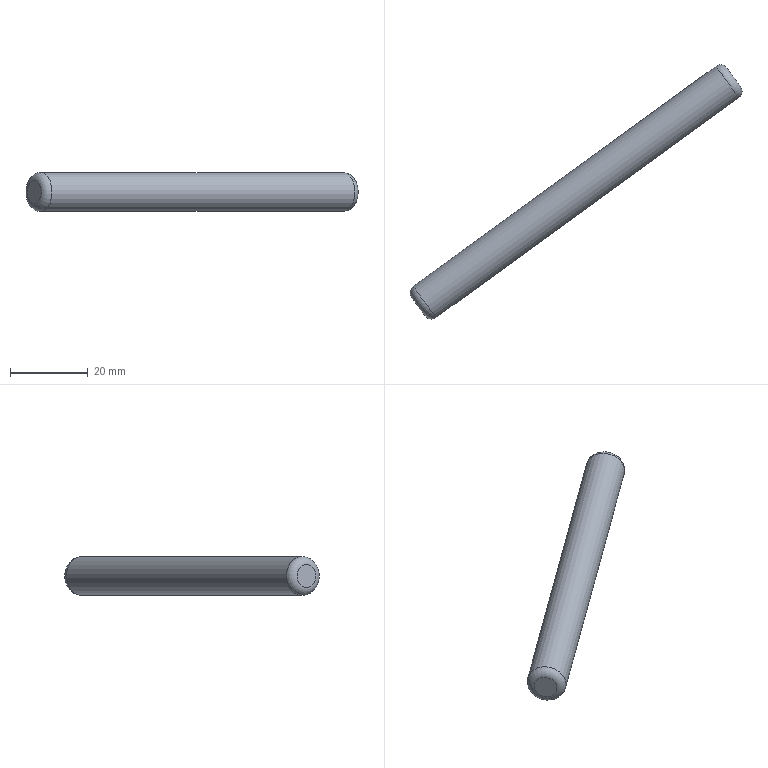Component | NX | CIBIK4 | 1 solid | 5 faces | box 85.19 x 65.28 x 10 mm | volume 7805 mm3 | plane 2 | torus 2 | cylinder 1 | commonest cylinder face diameters 10 x1
STEP:
#1=CARTESIAN_POINT('',(0.,0.,0.));
#2=DIRECTION('',(0.,0.,1.));
#3=DIRECTION('',(1.,0.,0.));
#4=AXIS2_PLACEMENT_3D('',#1,#2,#3);
#5=CARTESIAN_POINT('',(-1267.51,728.811,44.978));
#6=VERTEX_POINT('',#5);
#7=CARTESIAN_POINT('',(-1267.51,728.811,49.978));
#8=DIRECTION('',(0.809,0.5878,0.));
#9=DIRECTION('',(0.,0.,-1.));
#10=AXIS2_PLACEMENT_3D('',#7,#8,#9);
#11=CIRCLE('',#10,5.);
#12=CARTESIAN_POINT('',(-1188.227,786.414,49.978));
#13=DIRECTION('',(-0.809,-0.5878,0.));
#14=DIRECTION('',(0.,0.,1.));
#15=AXIS2_PLACEMENT_3D('',#12,#13,#14);
#16=CYLINDRICAL_SURFACE('',#15,5.);
#17=CARTESIAN_POINT('',(9.425,98.));
#18=DIRECTION('',(-1.,0.));
#19=VECTOR('',#18,1.);
#20=LINE('',#17,#19);
#21=(GEOMETRIC_REPRESENTATION_CONTEXT(2)PARAMETRIC_REPRESENTATION_CONTEXT()REPRESENTATION_CONTEXT('',''));
#22=DEFINITIONAL_REPRESENTATION('',(#20),#21);
#23=PCURVE('',#16,#22);
#24=CARTESIAN_POINT('',(-1267.51,728.811,49.978));
#25=DIRECTION('',(0.809,0.5878,0.));
#26=DIRECTION('',(0.,0.,-1.));
#27=AXIS2_PLACEMENT_3D('',#24,#25,#26);
#28=TOROIDAL_SURFACE('',#27,3.,2.);
#29=CARTESIAN_POINT('',(0.,6.283));
#30=DIRECTION('',(1.,0.));
#31=VECTOR('',#30,1.);
#32=LINE('',#29,#31);
#33=(GEOMETRIC_REPRESENTATION_CONTEXT(2)PARAMETRIC_REPRESENTATION_CONTEXT()REPRESENTATION_CONTEXT('',''));
#34=DEFINITIONAL_REPRESENTATION('',(#32),#33);
#35=PCURVE('',#28,#34);
#36=SURFACE_CURVE('',#11,(#23,#35),.PCURVE_S1.);
#37=EDGE_CURVE('',#6,#6,#36,.T.);
#38=ORIENTED_EDGE('',*,*,#37,.T.);
#39=CARTESIAN_POINT('',(-1189.845,785.238,44.978));
#40=VERTEX_POINT('',#39);
#41=CARTESIAN_POINT('',(-1189.845,785.238,44.978));
#42=CARTESIAN_POINT('',(-1267.51,728.811,44.978));
#43=B_SPLINE_CURVE_WITH_KNOTS('',1,(#41,#42),.UNSPECIFIED.,.F.,.F.,(2,2),(2.,98.),.PIECEWISE_BEZIER_KNOTS.);
#44=CARTESIAN_POINT('',(3.142,0.));
#45=DIRECTION('',(0.,1.));
#46=VECTOR('',#45,1.);
#47=LINE('',#44,#46);
#48=(GEOMETRIC_REPRESENTATION_CONTEXT(2)PARAMETRIC_REPRESENTATION_CONTEXT()REPRESENTATION_CONTEXT('',''));
#49=DEFINITIONAL_REPRESENTATION('',(#47),#48);
#50=PCURVE('',#16,#49);
#51=CARTESIAN_POINT('',(9.425,0.));
#52=DIRECTION('',(0.,1.));
#53=VECTOR('',#52,1.);
#54=LINE('',#51,#53);
#55=(GEOMETRIC_REPRESENTATION_CONTEXT(2)PARAMETRIC_REPRESENTATION_CONTEXT()REPRESENTATION_CONTEXT('',''));
#56=DEFINITIONAL_REPRESENTATION('',(#54),#55);
#57=PCURVE('',#16,#56);
#58=SEAM_CURVE('',#43,(#50,#57),.PCURVE_S1.);
#59=EDGE_CURVE('',#40,#6,#58,.T.);
#60=ORIENTED_EDGE('',*,*,#59,.F.);
#61=CARTESIAN_POINT('',(-1189.845,785.238,49.978));
#62=DIRECTION('',(-0.809,-0.5878,0.));
#63=DIRECTION('',(0.,0.,-1.));
#64=AXIS2_PLACEMENT_3D('',#61,#62,#63);
#65=CIRCLE('',#64,5.);
#66=CARTESIAN_POINT('',(3.142,2.));
#67=DIRECTION('',(1.,0.));
#68=VECTOR('',#67,1.);
#69=LINE('',#66,#68);
#70=(GEOMETRIC_REPRESENTATION_CONTEXT(2)PARAMETRIC_REPRESENTATION_CONTEXT()REPRESENTATION_CONTEXT('',''));
#71=DEFINITIONAL_REPRESENTATION('',(#69),#70);
#72=PCURVE('',#16,#71);
#73=CARTESIAN_POINT('',(-1189.845,785.238,49.978));
#74=DIRECTION('',(0.809,0.5878,0.));
#75=DIRECTION('',(0.,0.,-1.));
#76=AXIS2_PLACEMENT_3D('',#73,#74,#75);
#77=TOROIDAL_SURFACE('',#76,3.,2.);
#78=CARTESIAN_POINT('',(6.283,6.283));
#79=CARTESIAN_POINT('',(6.188,6.283));
#80=CARTESIAN_POINT('',(5.998,6.283));
#81=CARTESIAN_POINT('',(5.712,6.283));
#82=CARTESIAN_POINT('',(5.426,6.283));
#83=CARTESIAN_POINT('',(5.141,6.283));
#84=CARTESIAN_POINT('',(4.855,6.283));
#85=CARTESIAN_POINT('',(4.57,6.283));
#86=CARTESIAN_POINT('',(4.284,6.283));
#87=CARTESIAN_POINT('',(3.998,6.283));
#88=CARTESIAN_POINT('',(3.713,6.283));
#89=CARTESIAN_POINT('',(3.427,6.283));
#90=CARTESIAN_POINT('',(3.142,6.283));
#91=CARTESIAN_POINT('',(2.856,6.283));
#92=CARTESIAN_POINT('',(2.57,6.283));
#93=CARTESIAN_POINT('',(2.285,6.283));
#94=CARTESIAN_POINT('',(1.999,6.283));
#95=CARTESIAN_POINT('',(1.714,6.283));
#96=CARTESIAN_POINT('',(1.428,6.283));
#97=CARTESIAN_POINT('',(1.142,6.283));
#98=CARTESIAN_POINT('',(0.8568,6.283));
#99=CARTESIAN_POINT('',(0.5712,6.283));
#100=CARTESIAN_POINT('',(0.2856,6.283));
#101=CARTESIAN_POINT('',(0.0952,6.283));
#102=CARTESIAN_POINT('',(-0.,6.283));
#103=B_SPLINE_CURVE_WITH_KNOTS('',3,(#78,#79,#80,#81,#82,#83,#84,#85,#86,#87,#88,#89,#90,#91,#92,#93,#94,#95,#96,#97,#98,#99,#100,#101,#102),.UNSPECIFIED.,.F.,.F.,(4,1,1,1,1,1,1,1,1,1,1,1,1,1,1,1,1,1,1,1,1,1,4),(0.,0.2856,0.5712,0.8568,1.142,1.428,1.714,1.999,2.285,2.57,2.856,3.142,3.427,3.713,3.998,4.284,4.57,4.855,5.141,5.426,5.712,5.998,6.283),.QUASI_UNIFORM_KNOTS.);
#104=(GEOMETRIC_REPRESENTATION_CONTEXT(2)PARAMETRIC_REPRESENTATION_CONTEXT()REPRESENTATION_CONTEXT('',''));
#105=DEFINITIONAL_REPRESENTATION('',(#103),#104);
#106=PCURVE('',#77,#105);
#107=SURFACE_CURVE('',#65,(#72,#106),.PCURVE_S1.);
#108=EDGE_CURVE('',#40,#40,#107,.T.);
#109=ORIENTED_EDGE('',*,*,#108,.T.);
#110=ORIENTED_EDGE('',*,*,#59,.T.);
#111=EDGE_LOOP('',(#38,#60,#109,#110));
#112=FACE_BOUND('',#111,.T.);
#113=ADVANCED_FACE('',(#112),#16,.T.);
#114=CARTESIAN_POINT('',(-1188.227,786.414,46.978));
#115=VERTEX_POINT('',#114);
#116=CARTESIAN_POINT('',(-1188.227,786.414,49.978));
#117=DIRECTION('',(0.809,0.5878,0.));
#118=DIRECTION('',(0.,0.,-1.));
#119=AXIS2_PLACEMENT_3D('',#116,#117,#118);
#120=CIRCLE('',#119,3.);
#121=CARTESIAN_POINT('',(-1188.227,786.414,49.978));
#122=DIRECTION('',(0.809,0.5878,0.));
#123=DIRECTION('',(0.,0.,-1.));
#124=AXIS2_PLACEMENT_3D('',#121,#122,#123);
#125=PLANE('',#124);
#126=CARTESIAN_POINT('',(0.,0.));
#127=DIRECTION('',(1.,0.));
#128=AXIS2_PLACEMENT_2D('',#126,#127);
#129=CIRCLE('',#128,3.);
#130=(GEOMETRIC_REPRESENTATION_CONTEXT(2)PARAMETRIC_REPRESENTATION_CONTEXT()REPRESENTATION_CONTEXT('',''));
#131=DEFINITIONAL_REPRESENTATION('',(#129),#130);
#132=PCURVE('',#125,#131);
#133=CARTESIAN_POINT('',(0.,7.854));
#134=DIRECTION('',(1.,0.));
#135=VECTOR('',#134,1.);
#136=LINE('',#133,#135);
#137=(GEOMETRIC_REPRESENTATION_CONTEXT(2)PARAMETRIC_REPRESENTATION_CONTEXT()REPRESENTATION_CONTEXT('',''));
#138=DEFINITIONAL_REPRESENTATION('',(#136),#137);
#139=PCURVE('',#77,#138);
#140=SURFACE_CURVE('',#120,(#132,#139),.PCURVE_S1.);
#141=EDGE_CURVE('',#115,#115,#140,.T.);
#142=ORIENTED_EDGE('',*,*,#141,.T.);
#143=EDGE_LOOP('',(#142));
#144=FACE_BOUND('',#143,.T.);
#145=ADVANCED_FACE('',(#144),#125,.T.);
#146=CARTESIAN_POINT('',(-1269.128,727.635,46.978));
#147=VERTEX_POINT('',#146);
#148=CARTESIAN_POINT('',(-1269.128,727.635,49.978));
#149=DIRECTION('',(-0.809,-0.5878,0.));
#150=DIRECTION('',(0.,0.,-1.));
#151=AXIS2_PLACEMENT_3D('',#148,#149,#150);
#152=CIRCLE('',#151,3.);
#153=CARTESIAN_POINT('',(-1269.128,727.635,49.978));
#154=DIRECTION('',(0.809,0.5878,0.));
#155=DIRECTION('',(0.,0.,-1.));
#156=AXIS2_PLACEMENT_3D('',#153,#154,#155);
#157=PLANE('',#156);
#158=CARTESIAN_POINT('',(3.,0.));
#159=CARTESIAN_POINT('',(3.,-5.196));
#160=CARTESIAN_POINT('',(-1.5,-2.598));
#161=CARTESIAN_POINT('',(-6.,-0.));
#162=CARTESIAN_POINT('',(-1.5,2.598));
#163=CARTESIAN_POINT('',(3.,5.196));
#164=CARTESIAN_POINT('',(3.,0.));
#165=(BOUNDED_CURVE()B_SPLINE_CURVE(2,(#158,#159,#160,#161,#162,#163,#164),.UNSPECIFIED.,.T.,.F.)B_SPLINE_CURVE_WITH_KNOTS((1,2,2,2,2,1),(-2.094,0.,2.094,4.189,6.283,8.378),.UNSPECIFIED.)CURVE()GEOMETRIC_REPRESENTATION_ITEM()RATIONAL_B_SPLINE_CURVE((1.,0.5,1.,0.5,1.,0.5,1.))REPRESENTATION_ITEM(''));
#166=(GEOMETRIC_REPRESENTATION_CONTEXT(2)PARAMETRIC_REPRESENTATION_CONTEXT()REPRESENTATION_CONTEXT('',''));
#167=DEFINITIONAL_REPRESENTATION('',(#165),#166);
#168=PCURVE('',#157,#167);
#169=CARTESIAN_POINT('',(6.283,4.712));
#170=DIRECTION('',(-1.,0.));
#171=VECTOR('',#170,1.);
#172=LINE('',#169,#171);
#173=(GEOMETRIC_REPRESENTATION_CONTEXT(2)PARAMETRIC_REPRESENTATION_CONTEXT()REPRESENTATION_CONTEXT('',''));
#174=DEFINITIONAL_REPRESENTATION('',(#172),#173);
#175=PCURVE('',#28,#174);
#176=SURFACE_CURVE('',#152,(#168,#175),.PCURVE_S1.);
#177=EDGE_CURVE('',#147,#147,#176,.T.);
#178=ORIENTED_EDGE('',*,*,#177,.T.);
#179=EDGE_LOOP('',(#178));
#180=FACE_BOUND('',#179,.T.);
#181=ADVANCED_FACE('',(#180),#157,.F.);
#182=ORIENTED_EDGE('',*,*,#177,.F.);
#183=CARTESIAN_POINT('',(-1269.128,727.635,46.978));
#184=CARTESIAN_POINT('',(-1269.128,727.635,46.443));
#185=CARTESIAN_POINT('',(-1268.991,727.735,45.922));
#186=CARTESIAN_POINT('',(-1268.727,727.927,45.474));
#187=CARTESIAN_POINT('',(-1268.364,728.191,45.148));
#188=CARTESIAN_POINT('',(-1267.943,728.497,44.978));
#189=CARTESIAN_POINT('',(-1267.51,728.811,44.978));
#190=(BOUNDED_CURVE()B_SPLINE_CURVE(6,(#183,#184,#185,#186,#187,#188,#189),.UNSPECIFIED.,.F.,.F.)B_SPLINE_CURVE_WITH_KNOTS((7,7),(4.712,6.283),.PIECEWISE_BEZIER_KNOTS.)CURVE()GEOMETRIC_REPRESENTATION_ITEM()RATIONAL_B_SPLINE_CURVE((1.031,1.01,0.9979,0.994,0.9979,1.01,1.031))REPRESENTATION_ITEM(''));
#191=CARTESIAN_POINT('',(6.283,0.));
#192=DIRECTION('',(0.,1.));
#193=VECTOR('',#192,1.);
#194=LINE('',#191,#193);
#195=(GEOMETRIC_REPRESENTATION_CONTEXT(2)PARAMETRIC_REPRESENTATION_CONTEXT()REPRESENTATION_CONTEXT('',''));
#196=DEFINITIONAL_REPRESENTATION('',(#194),#195);
#197=PCURVE('',#28,#196);
#198=CARTESIAN_POINT('',(0.,0.));
#199=DIRECTION('',(0.,1.));
#200=VECTOR('',#199,1.);
#201=LINE('',#198,#200);
#202=(GEOMETRIC_REPRESENTATION_CONTEXT(2)PARAMETRIC_REPRESENTATION_CONTEXT()REPRESENTATION_CONTEXT('',''));
#203=DEFINITIONAL_REPRESENTATION('',(#201),#202);
#204=PCURVE('',#28,#203);
#205=SEAM_CURVE('',#190,(#197,#204),.PCURVE_S1.);
#206=EDGE_CURVE('',#147,#6,#205,.T.);
#207=ORIENTED_EDGE('',*,*,#206,.T.);
#208=ORIENTED_EDGE('',*,*,#37,.F.);
#209=ORIENTED_EDGE('',*,*,#206,.F.);
#210=EDGE_LOOP('',(#182,#207,#208,#209));
#211=FACE_BOUND('',#210,.T.);
#212=ADVANCED_FACE('',(#211),#28,.T.);
#213=ORIENTED_EDGE('',*,*,#108,.F.);
#214=CARTESIAN_POINT('',(-1189.845,785.238,44.978));
#215=CARTESIAN_POINT('',(-1189.412,785.553,44.978));
#216=CARTESIAN_POINT('',(-1188.991,785.859,45.148));
#217=CARTESIAN_POINT('',(-1188.628,786.122,45.474));
#218=CARTESIAN_POINT('',(-1188.364,786.314,45.922));
#219=CARTESIAN_POINT('',(-1188.227,786.414,46.443));
#220=CARTESIAN_POINT('',(-1188.227,786.414,46.978));
#221=(BOUNDED_CURVE()B_SPLINE_CURVE(6,(#214,#215,#216,#217,#218,#219,#220),.UNSPECIFIED.,.F.,.F.)B_SPLINE_CURVE_WITH_KNOTS((7,7),(6.283,7.854),.PIECEWISE_BEZIER_KNOTS.)CURVE()GEOMETRIC_REPRESENTATION_ITEM()RATIONAL_B_SPLINE_CURVE((1.031,1.01,0.9979,0.994,0.9979,1.01,1.031))REPRESENTATION_ITEM(''));
#222=CARTESIAN_POINT('',(6.283,0.));
#223=DIRECTION('',(0.,1.));
#224=VECTOR('',#223,1.);
#225=LINE('',#222,#224);
#226=(GEOMETRIC_REPRESENTATION_CONTEXT(2)PARAMETRIC_REPRESENTATION_CONTEXT()REPRESENTATION_CONTEXT('',''));
#227=DEFINITIONAL_REPRESENTATION('',(#225),#226);
#228=PCURVE('',#77,#227);
#229=CARTESIAN_POINT('',(0.,0.));
#230=DIRECTION('',(0.,1.));
#231=VECTOR('',#230,1.);
#232=LINE('',#229,#231);
#233=(GEOMETRIC_REPRESENTATION_CONTEXT(2)PARAMETRIC_REPRESENTATION_CONTEXT()REPRESENTATION_CONTEXT('',''));
#234=DEFINITIONAL_REPRESENTATION('',(#232),#233);
#235=PCURVE('',#77,#234);
#236=SEAM_CURVE('',#221,(#228,#235),.PCURVE_S1.);
#237=EDGE_CURVE('',#40,#115,#236,.T.);
#238=ORIENTED_EDGE('',*,*,#237,.T.);
#239=ORIENTED_EDGE('',*,*,#141,.F.);
#240=ORIENTED_EDGE('',*,*,#237,.F.);
#241=EDGE_LOOP('',(#213,#238,#239,#240));
#242=FACE_BOUND('',#241,.T.);
#243=ADVANCED_FACE('',(#242),#77,.T.);
#244=CLOSED_SHELL('',(#113,#145,#181,#212,#243));
#245=MANIFOLD_SOLID_BREP('',#244);
#246=(LENGTH_UNIT()NAMED_UNIT(*)SI_UNIT(.MILLI.,.METRE.));
#247=UNCERTAINTY_MEASURE_WITH_UNIT(LENGTH_MEASURE(0.00001),#246,'','');
#248=(NAMED_UNIT(*)PLANE_ANGLE_UNIT()SI_UNIT($,.RADIAN.));
#249=(NAMED_UNIT(*)SI_UNIT($,.STERADIAN.)SOLID_ANGLE_UNIT());
#250=(GEOMETRIC_REPRESENTATION_CONTEXT(3)GLOBAL_UNCERTAINTY_ASSIGNED_CONTEXT((#247))GLOBAL_UNIT_ASSIGNED_CONTEXT((#246,#248,#249))REPRESENTATION_CONTEXT('',''));
#251=ADVANCED_BREP_SHAPE_REPRESENTATION('',(#4,#245),#250);